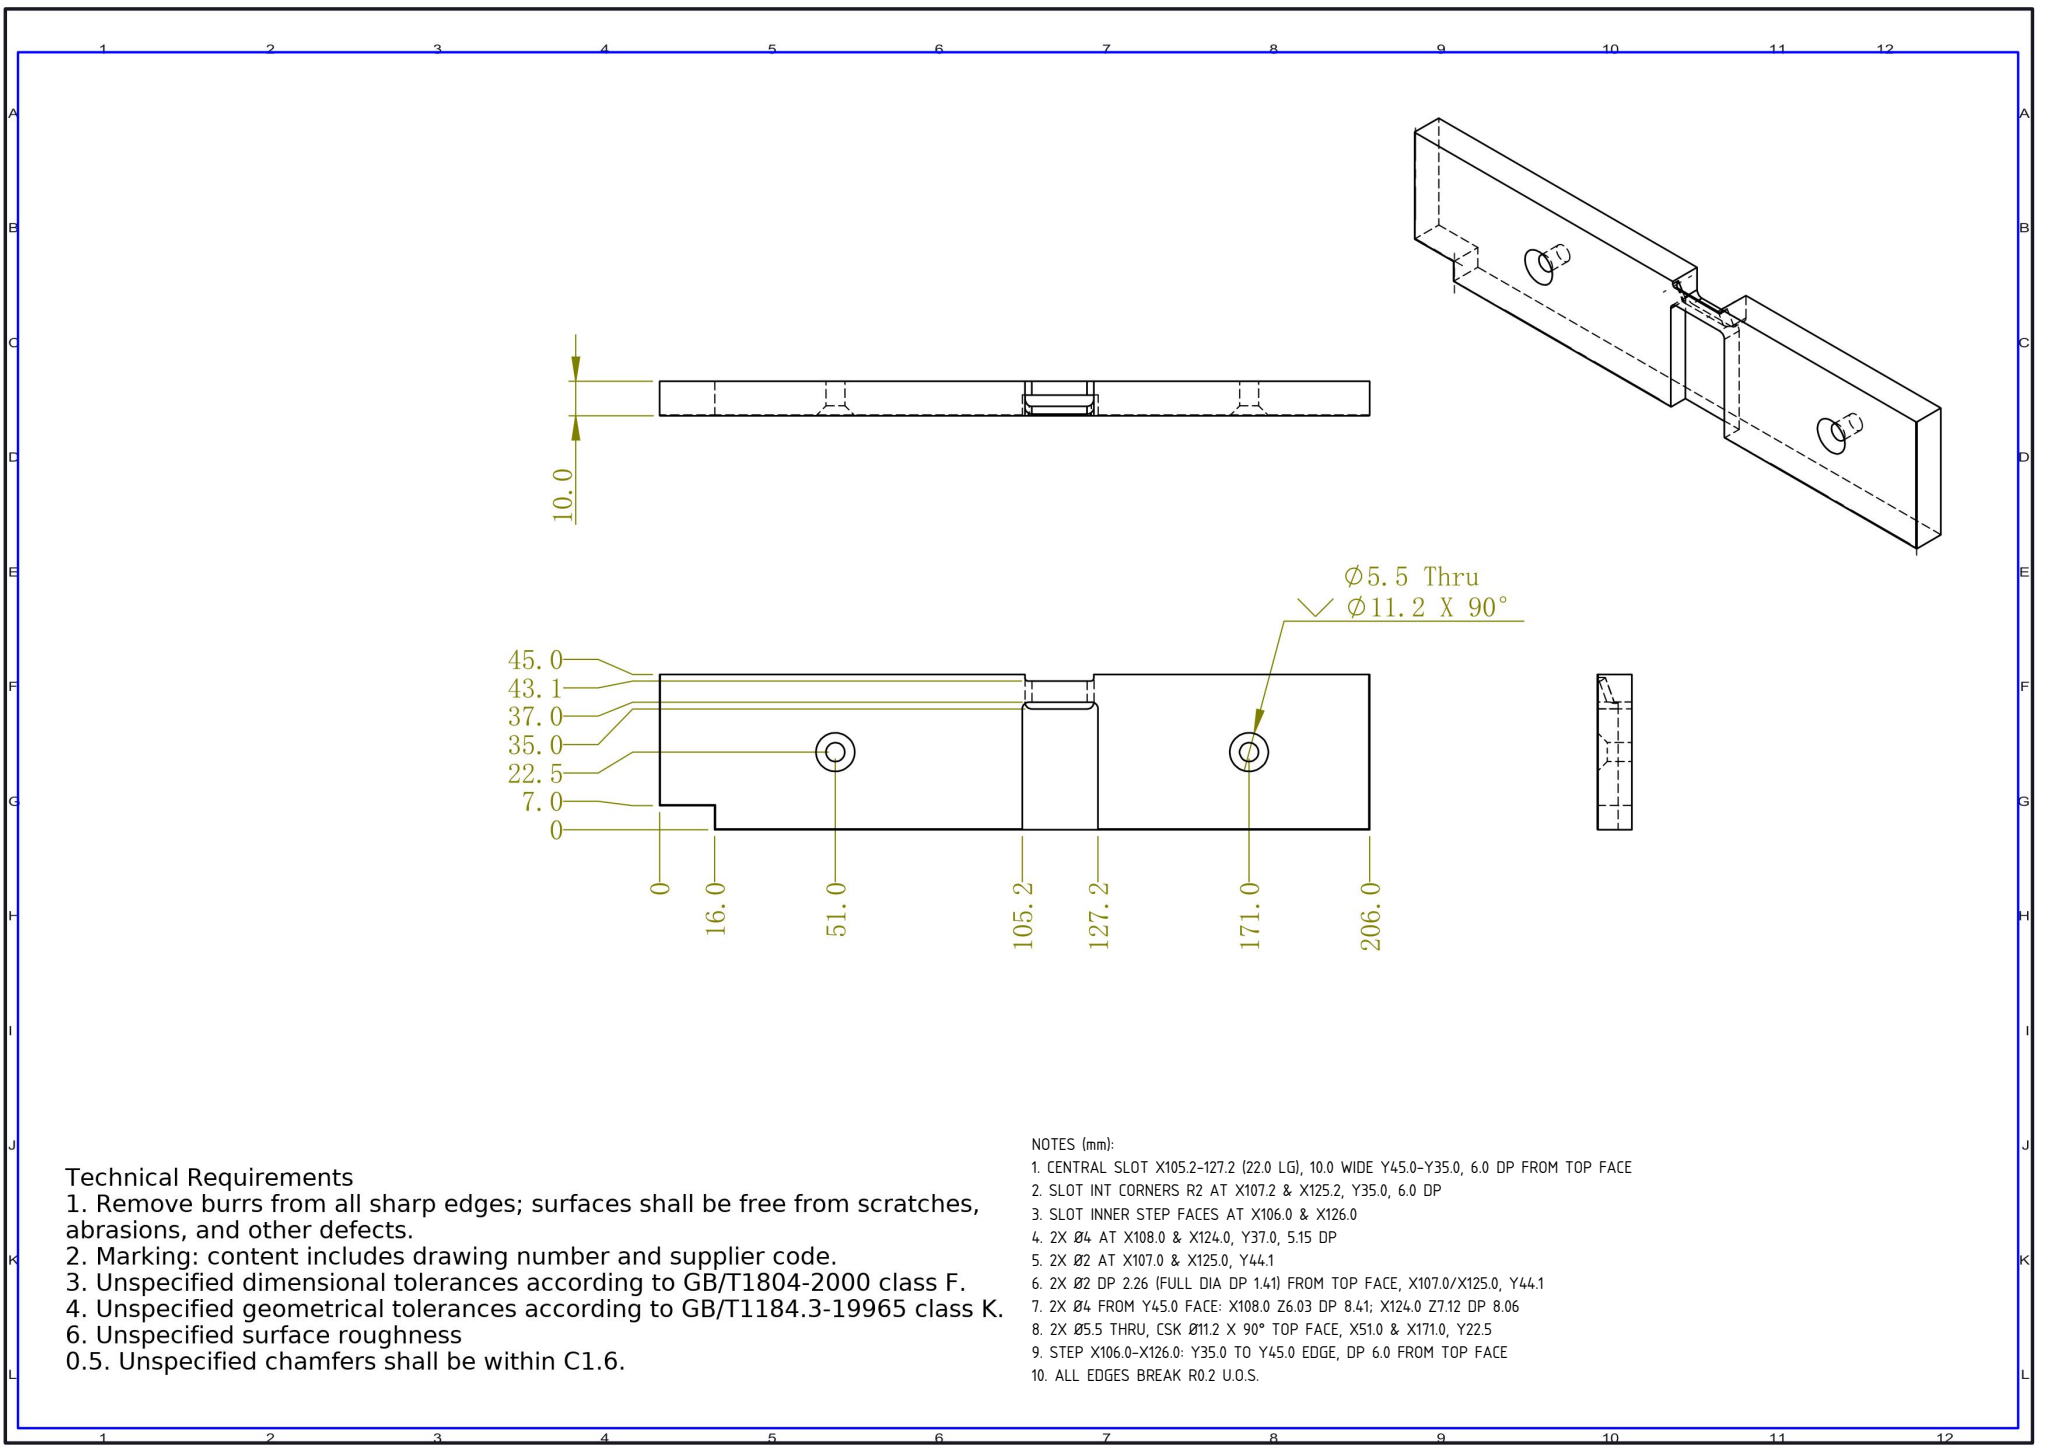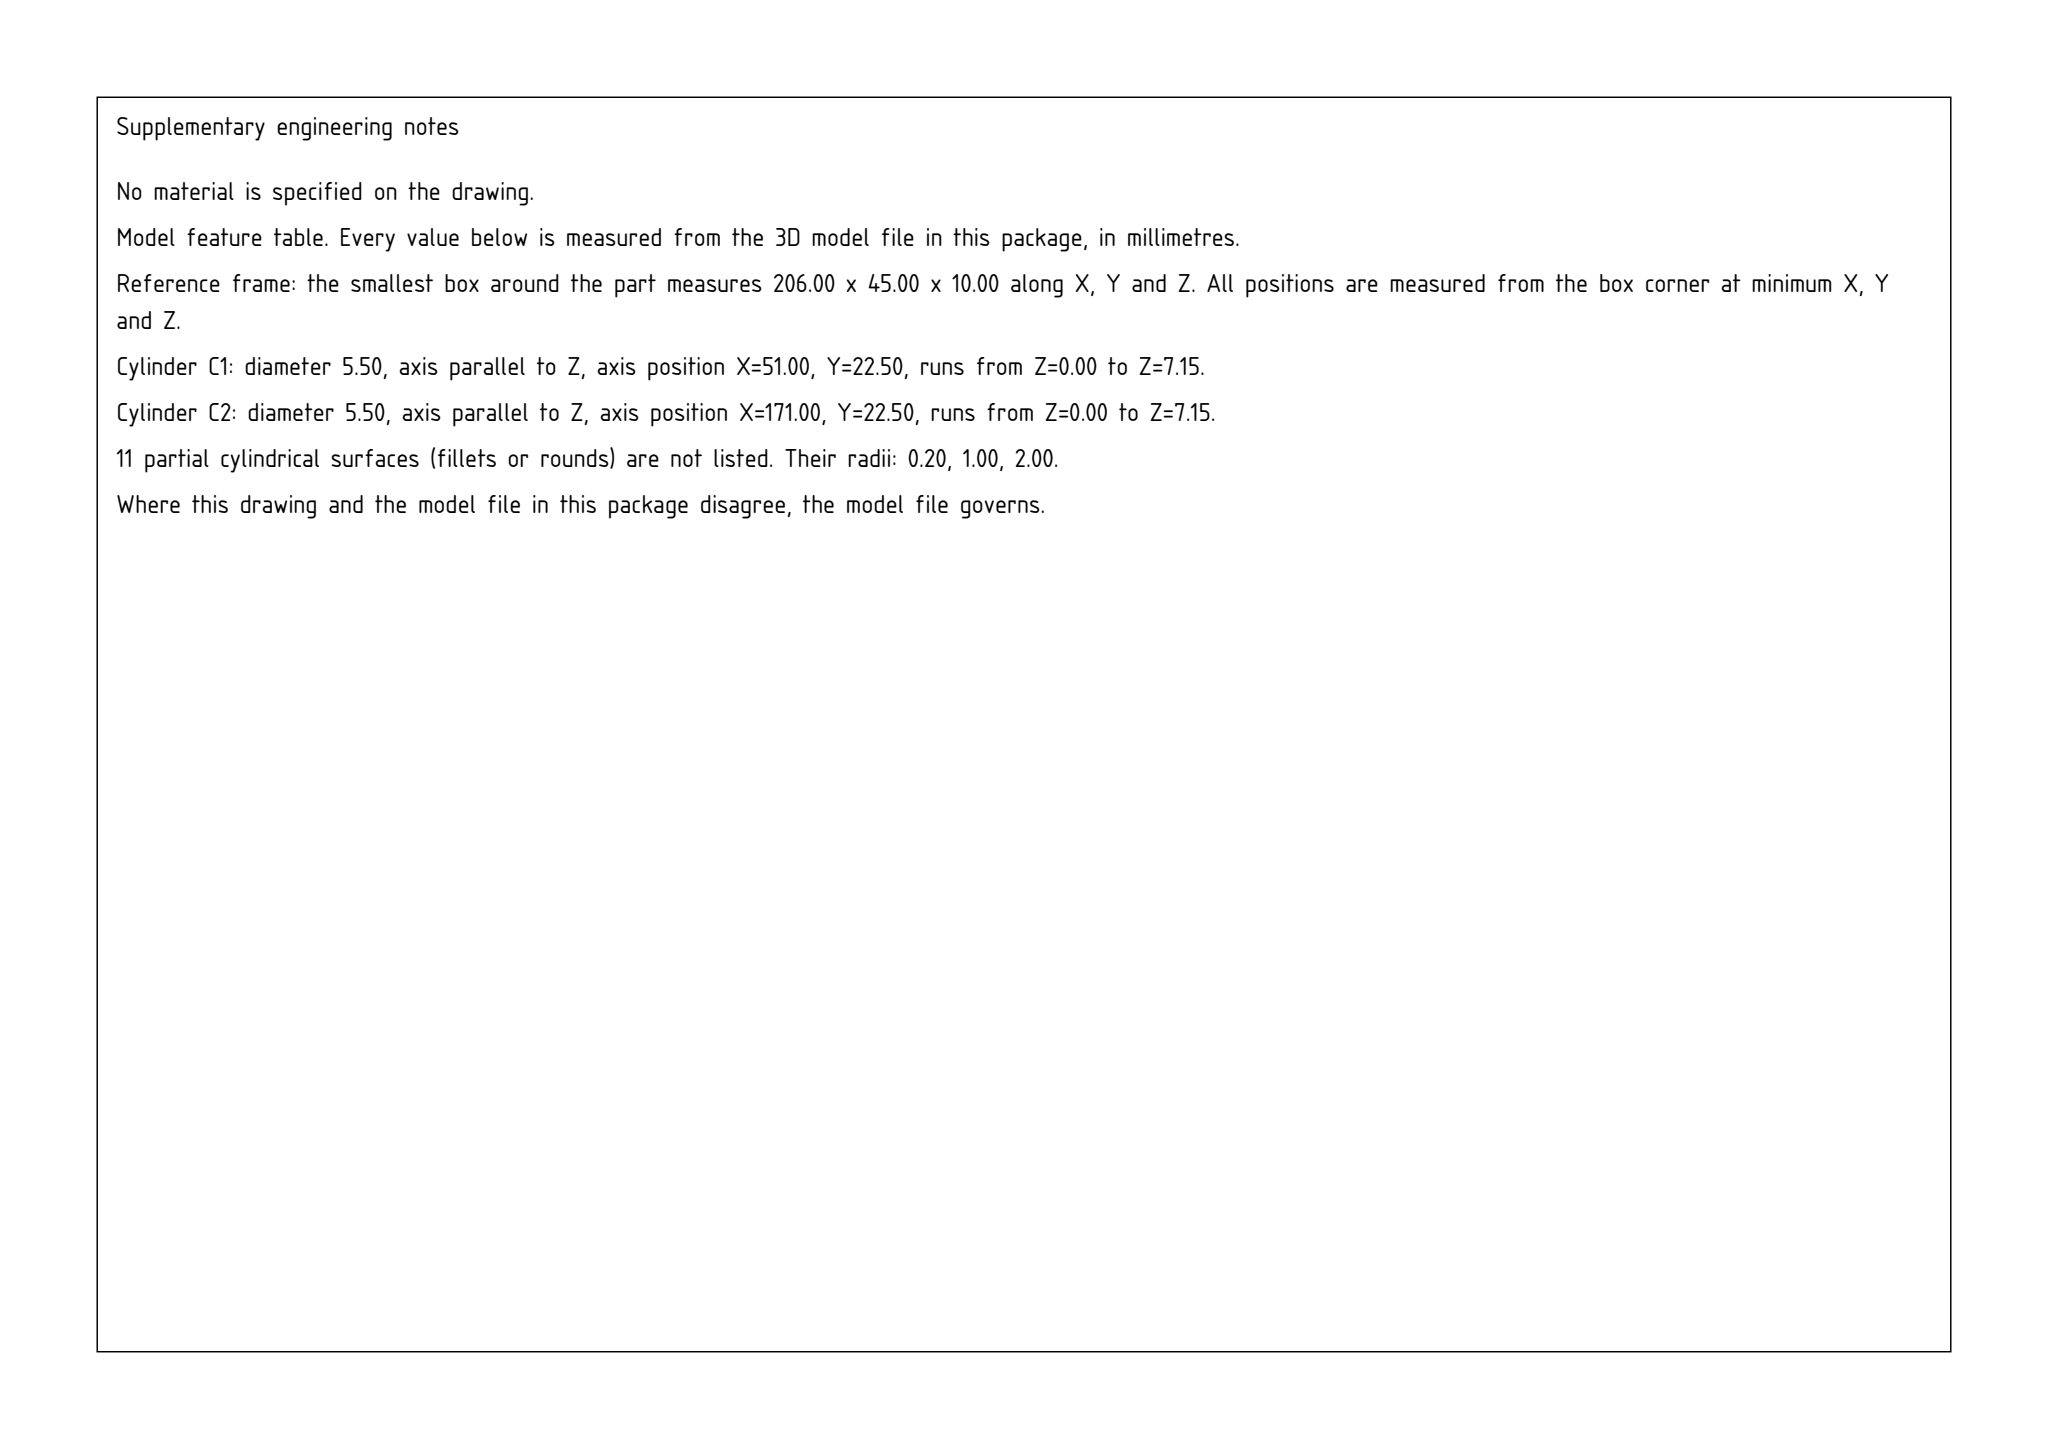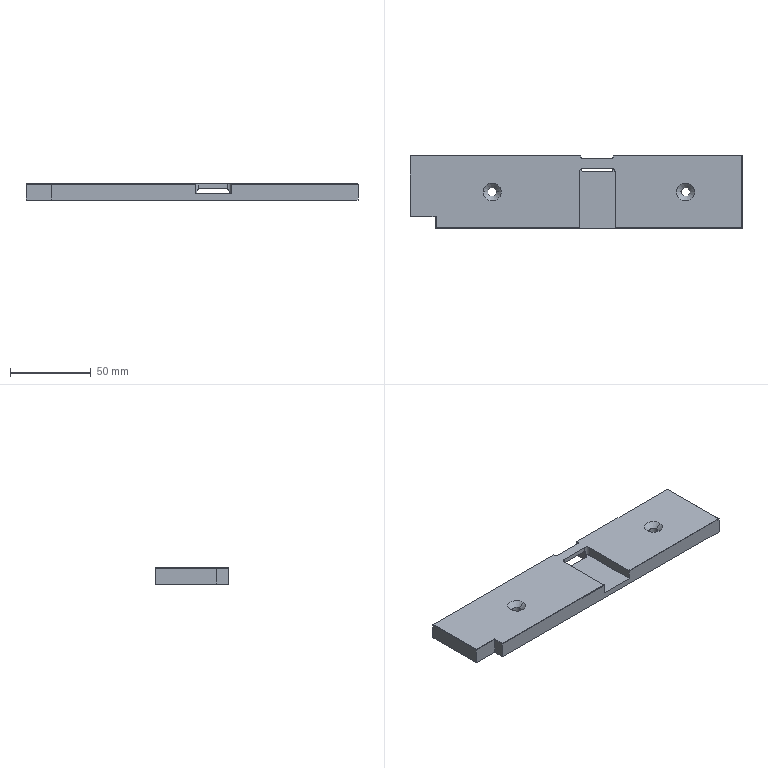Part | SolidWorks | mm | 1 solid | 48 faces | box 206 x 45 x 10 mm | volume 84495 mm3 | cylinder 26 | plane 18 | cone 4 | commonest cylinder face diameters 0.4 x12 4 x6 5.5 x4 2 x4
Drawing notes:
CENTRAL SLOT X105.2-127.2 (22.0 LG), 10.0 WIDE Y45.0-Y35.0, 6.0 DP FROM TOP FACE | from the solid: x planes 105.2 & 127.2; y planes 45.0 & 35.0; z planes 10.0 & 4.0 = 6.0 DP
SLOT INT CORNERS R2 AT X107.2 & X125.2, Y35.0, 6.0 DP | from the solid: Ø4 z-axis cyls at (107.2,35.0) and (125.2,35.0), L=6.0 (Z10 to Z4)
SLOT INNER STEP FACES AT X106.0 & X126.0 | from the solid: axis planes normal x at offsets 106.0 and 126.0
2X Ø4 AT X108.0 & X124.0, Y37.0, 5.15 DP | from the solid: Ø4 z-axis cyls at (108.0,37.0) & (124.0,37.0), L=5.15
2X Ø2 AT X107.0 & X125.0, Y44.1 | from the solid: Ø2 z-axis cyls at (107.0,44.1) & (125.0,44.1)
2X Ø2 DP 2.26 (FULL DIA DP 1.41) FROM TOP FACE, X107.0/X125.0, Y44.1 | from the solid: Ø2 z-axis cylinders at (107.0,44.1) and (125.0,44.1), L=1.41 & 2.26; top face z=10.0
2X Ø4 FROM Y45.0 FACE: X108.0 Z6.03 DP 8.41; X124.0 Z7.12 DP 8.06 | from the solid: Ø4 y-axis cylinders at x=108.0 z=6.03 L8.41 and x=124.0 z=7.12 L8.06; y face plane at 45.0 (45-8.41=36.59, 45-8.06=36.94)
2X Ø5.5 THRU, CSK Ø11.2 X 90° TOP FACE, X51.0 & X171.0, Y22.5 | from the solid: Ø5.5 z-axis cylinders at (51.0,22.5) and (171.0,22.5) L7.15 in 10 thk; cones 90° ref dia 11.2 (7.15+2.85=10)
STEP X106.0-X126.0: Y35.0 TO Y45.0 EDGE, DP 6.0 FROM TOP FACE | from the solid: x-planes 106.0 & 126.0; y-planes 35.0 & 45.0; z-planes 10.0 top and 4.0 floor (6.0 deep); R2 corner cyls dia4 at (108,37) & (124,37) tangent to x106/y35, 6.0 long
ALL EDGES BREAK R0.2 U.O.S. | from the solid: dia 0.4 edge-blend cylinders along x,y edges at offsets 0.2 from faces (y0.2/z9.8, x0.2, x205.8, x16.2, y7.2)